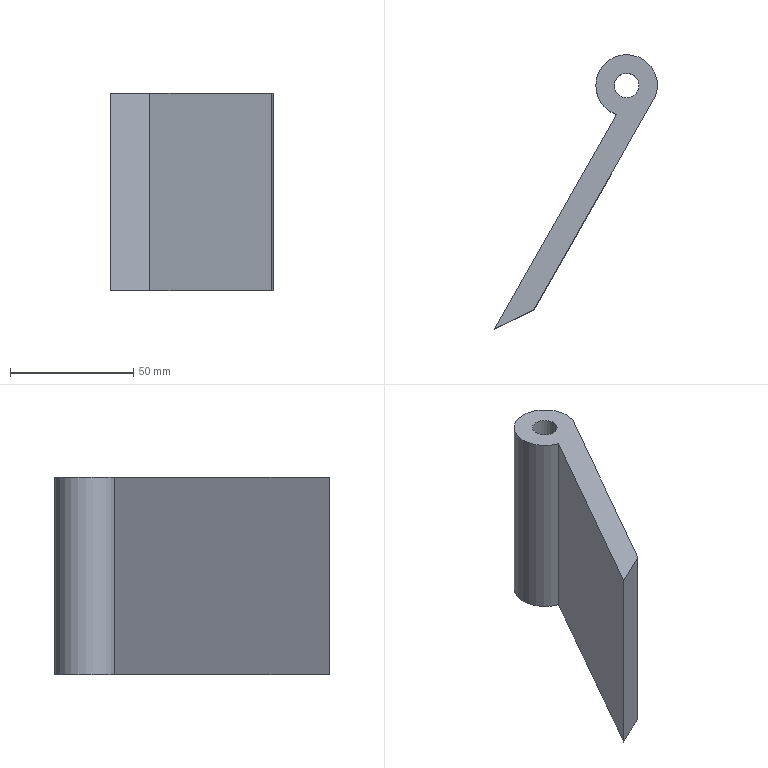Component | SolidWorks | Scraper-1 | 1 solid | 8 faces | box 66.03 x 111.24 x 80 mm | volume 109419 mm3 | plane 5 | cylinder 3 | commonest cylinder face diameters 10 x2 25 x1
build123d program:
from build123d import *

# Parameters (mm, degrees)
SKETCH1_R           = 5
BOSS_EXTRUDE1_DEPTH = 80


with BuildPart() as part:
    # Sketch1 → Boss-Extrude1 (new body)
    with BuildSketch(Plane(origin=(0, 0, 0), x_dir=(0, 0, -1), z_dir=(1, 0, 0))):
        with BuildLine():
            Line((-12.5, 0), (5.81, -98.31))
            Line((5.81, -98.31), (18.31, -110.81))
            Line((18.31, -110.81), (0, -12.5))
            ThreePointArc((0, -12.5), (8.839, 8.839), (-12.5, 0))
        make_face()
        Circle(SKETCH1_R, mode=Mode.SUBTRACT)
    extrude(amount=BOSS_EXTRUDE1_DEPTH)


solid = part.part

# Placed as in the assembly
solid = solid.moved(Location((504.241, -232.715, 1598.724), (90, 70.919, -90)))
STEP:
#1=COLOUR_RGB('',0.7922,0.8196,0.9333);
#2=FILL_AREA_STYLE_COLOUR('',#1);
#3=FILL_AREA_STYLE('',(#2));
#4=SURFACE_STYLE_FILL_AREA(#3);
#5=SURFACE_SIDE_STYLE('',(#4));
#6=SURFACE_STYLE_USAGE(.BOTH.,#5);
#7=PRESENTATION_STYLE_ASSIGNMENT((#6));
#8=CARTESIAN_POINT('',(20.038,-9.226,59.792));
#9=VERTEX_POINT('',#8);
#10=CARTESIAN_POINT('',(19.666,-9.098,59.792));
#11=VERTEX_POINT('',#10);
#12=CARTESIAN_POINT('',(19.852,-9.162,59.792));
#13=DIRECTION('',(-0.,-0.,-1.));
#14=DIRECTION('',(-0.9451,0.3269,0.));
#15=AXIS2_PLACEMENT_3D('',#12,#13,#14);
#16=CIRCLE('',#15,0.1969);
#17=EDGE_CURVE('',#9,#11,#16,.T.);
#18=ORIENTED_EDGE('',*,*,#17,.T.);
#19=CARTESIAN_POINT('',(19.666,-9.098,62.942));
#20=VERTEX_POINT('',#19);
#21=CARTESIAN_POINT('',(19.666,-9.098,59.792));
#22=DIRECTION('',(0.,0.,1.));
#23=VECTOR('',#22,39.37);
#24=LINE('',#21,#23);
#25=EDGE_CURVE('',#11,#20,#24,.T.);
#26=ORIENTED_EDGE('',*,*,#25,.T.);
#27=CARTESIAN_POINT('',(20.038,-9.226,62.942));
#28=VERTEX_POINT('',#27);
#29=CARTESIAN_POINT('',(19.852,-9.162,62.942));
#30=DIRECTION('',(-0.,-0.,-1.));
#31=DIRECTION('',(-0.9451,0.3269,0.));
#32=AXIS2_PLACEMENT_3D('',#29,#30,#31);
#33=CIRCLE('',#32,0.1969);
#34=EDGE_CURVE('',#28,#20,#33,.T.);
#35=ORIENTED_EDGE('',*,*,#34,.F.);
#36=CARTESIAN_POINT('',(20.038,-9.226,59.792));
#37=DIRECTION('',(0.,0.,1.));
#38=VECTOR('',#37,39.37);
#39=LINE('',#36,#38);
#40=EDGE_CURVE('',#9,#28,#39,.T.);
#41=ORIENTED_EDGE('',*,*,#40,.F.);
#42=EDGE_LOOP('',(#18,#26,#35,#41));
#43=FACE_OUTER_BOUND('',#42,.T.);
#44=CARTESIAN_POINT('',(19.852,-9.162,59.792));
#45=DIRECTION('',(0.,0.,1.));
#46=DIRECTION('',(0.9451,-0.3269,0.));
#47=AXIS2_PLACEMENT_3D('',#44,#45,#46);
#48=CYLINDRICAL_SURFACE('',#47,0.1969);
#49=ADVANCED_FACE('',(#43),#48,.F.);
#50=CARTESIAN_POINT('',(19.691,-9.627,59.792));
#51=VERTEX_POINT('',#50);
#52=CARTESIAN_POINT('',(20.317,-9.323,59.792));
#53=VERTEX_POINT('',#52);
#54=CARTESIAN_POINT('',(19.852,-9.162,59.792));
#55=DIRECTION('',(-0.,-0.,-1.));
#56=DIRECTION('',(-0.9451,0.3269,0.));
#57=AXIS2_PLACEMENT_3D('',#54,#55,#56);
#58=CIRCLE('',#57,0.4921);
#59=EDGE_CURVE('',#51,#53,#58,.T.);
#60=ORIENTED_EDGE('',*,*,#59,.T.);
#61=CARTESIAN_POINT('',(18.371,-12.745,59.792));
#62=VERTEX_POINT('',#61);
#63=CARTESIAN_POINT('',(20.317,-9.323,59.792));
#64=DIRECTION('',(-0.4944,-0.8692,0.));
#65=VECTOR('',#64,39.37);
#66=LINE('',#63,#65);
#67=EDGE_CURVE('',#53,#62,#66,.T.);
#68=ORIENTED_EDGE('',*,*,#67,.T.);
#69=CARTESIAN_POINT('',(17.745,-13.049,59.792));
#70=VERTEX_POINT('',#69);
#71=CARTESIAN_POINT('',(18.371,-12.745,59.792));
#72=DIRECTION('',(-0.8994,-0.4371,0.));
#73=VECTOR('',#72,39.37);
#74=LINE('',#71,#73);
#75=EDGE_CURVE('',#62,#70,#74,.T.);
#76=ORIENTED_EDGE('',*,*,#75,.T.);
#77=CARTESIAN_POINT('',(17.745,-13.049,59.792));
#78=DIRECTION('',(0.4944,0.8692,-0.));
#79=VECTOR('',#78,39.37);
#80=LINE('',#77,#79);
#81=EDGE_CURVE('',#70,#51,#80,.T.);
#82=ORIENTED_EDGE('',*,*,#81,.T.);
#83=EDGE_LOOP('',(#60,#68,#76,#82));
#84=FACE_OUTER_BOUND('',#83,.T.);
#85=ORIENTED_EDGE('',*,*,#17,.F.);
#86=CARTESIAN_POINT('',(19.852,-9.162,59.792));
#87=DIRECTION('',(-0.,-0.,-1.));
#88=DIRECTION('',(-0.9451,0.3269,0.));
#89=AXIS2_PLACEMENT_3D('',#86,#87,#88);
#90=CIRCLE('',#89,0.1969);
#91=EDGE_CURVE('',#11,#9,#90,.T.);
#92=ORIENTED_EDGE('',*,*,#91,.F.);
#93=EDGE_LOOP('',(#85,#92));
#94=FACE_BOUND('',#93,.T.);
#95=CARTESIAN_POINT('',(19.852,-9.162,59.792));
#96=DIRECTION('',(-0.,-0.,-1.));
#97=DIRECTION('',(-0.9451,0.3269,0.));
#98=AXIS2_PLACEMENT_3D('',#95,#96,#97);
#99=PLANE('',#98);
#100=ADVANCED_FACE('',(#84,#94),#99,.T.);
#101=CARTESIAN_POINT('',(19.691,-9.627,62.942));
#102=VERTEX_POINT('',#101);
#103=CARTESIAN_POINT('',(20.317,-9.323,62.942));
#104=VERTEX_POINT('',#103);
#105=CARTESIAN_POINT('',(19.852,-9.162,62.942));
#106=DIRECTION('',(-0.,-0.,-1.));
#107=DIRECTION('',(-0.9451,0.3269,0.));
#108=AXIS2_PLACEMENT_3D('',#105,#106,#107);
#109=CIRCLE('',#108,0.4921);
#110=EDGE_CURVE('',#102,#104,#109,.T.);
#111=ORIENTED_EDGE('',*,*,#110,.F.);
#112=CARTESIAN_POINT('',(17.745,-13.049,62.942));
#113=VERTEX_POINT('',#112);
#114=CARTESIAN_POINT('',(17.745,-13.049,62.942));
#115=DIRECTION('',(0.4944,0.8692,-0.));
#116=VECTOR('',#115,39.37);
#117=LINE('',#114,#116);
#118=EDGE_CURVE('',#113,#102,#117,.T.);
#119=ORIENTED_EDGE('',*,*,#118,.F.);
#120=CARTESIAN_POINT('',(18.371,-12.745,62.942));
#121=VERTEX_POINT('',#120);
#122=CARTESIAN_POINT('',(18.371,-12.745,62.942));
#123=DIRECTION('',(-0.8994,-0.4371,0.));
#124=VECTOR('',#123,39.37);
#125=LINE('',#122,#124);
#126=EDGE_CURVE('',#121,#113,#125,.T.);
#127=ORIENTED_EDGE('',*,*,#126,.F.);
#128=CARTESIAN_POINT('',(20.317,-9.323,62.942));
#129=DIRECTION('',(-0.4944,-0.8692,0.));
#130=VECTOR('',#129,39.37);
#131=LINE('',#128,#130);
#132=EDGE_CURVE('',#104,#121,#131,.T.);
#133=ORIENTED_EDGE('',*,*,#132,.F.);
#134=EDGE_LOOP('',(#111,#119,#127,#133));
#135=FACE_OUTER_BOUND('',#134,.T.);
#136=ORIENTED_EDGE('',*,*,#34,.T.);
#137=CARTESIAN_POINT('',(19.852,-9.162,62.942));
#138=DIRECTION('',(-0.,-0.,-1.));
#139=DIRECTION('',(-0.9451,0.3269,0.));
#140=AXIS2_PLACEMENT_3D('',#137,#138,#139);
#141=CIRCLE('',#140,0.1969);
#142=EDGE_CURVE('',#20,#28,#141,.T.);
#143=ORIENTED_EDGE('',*,*,#142,.T.);
#144=EDGE_LOOP('',(#136,#143));
#145=FACE_BOUND('',#144,.T.);
#146=CARTESIAN_POINT('',(19.852,-9.162,62.942));
#147=DIRECTION('',(-0.,-0.,-1.));
#148=DIRECTION('',(-0.9451,0.3269,0.));
#149=AXIS2_PLACEMENT_3D('',#146,#147,#148);
#150=PLANE('',#149);
#151=ADVANCED_FACE('',(#135,#145),#150,.F.);
#152=ORIENTED_EDGE('',*,*,#110,.T.);
#153=CARTESIAN_POINT('',(20.317,-9.323,59.792));
#154=DIRECTION('',(0.,0.,1.));
#155=VECTOR('',#154,39.37);
#156=LINE('',#153,#155);
#157=EDGE_CURVE('',#53,#104,#156,.T.);
#158=ORIENTED_EDGE('',*,*,#157,.F.);
#159=ORIENTED_EDGE('',*,*,#59,.F.);
#160=CARTESIAN_POINT('',(19.691,-9.627,59.792));
#161=DIRECTION('',(0.,0.,1.));
#162=VECTOR('',#161,39.37);
#163=LINE('',#160,#162);
#164=EDGE_CURVE('',#51,#102,#163,.T.);
#165=ORIENTED_EDGE('',*,*,#164,.T.);
#166=EDGE_LOOP('',(#152,#158,#159,#165));
#167=FACE_OUTER_BOUND('',#166,.T.);
#168=CARTESIAN_POINT('',(19.852,-9.162,59.792));
#169=DIRECTION('',(0.,0.,1.));
#170=DIRECTION('',(0.9451,-0.3269,0.));
#171=AXIS2_PLACEMENT_3D('',#168,#169,#170);
#172=CYLINDRICAL_SURFACE('',#171,0.4921);
#173=ADVANCED_FACE('',(#167),#172,.T.);
#174=ORIENTED_EDGE('',*,*,#132,.T.);
#175=CARTESIAN_POINT('',(18.371,-12.745,59.792));
#176=DIRECTION('',(0.,0.,1.));
#177=VECTOR('',#176,39.37);
#178=LINE('',#175,#177);
#179=EDGE_CURVE('',#62,#121,#178,.T.);
#180=ORIENTED_EDGE('',*,*,#179,.F.);
#181=ORIENTED_EDGE('',*,*,#67,.F.);
#182=ORIENTED_EDGE('',*,*,#157,.T.);
#183=EDGE_LOOP('',(#174,#180,#181,#182));
#184=FACE_OUTER_BOUND('',#183,.T.);
#185=CARTESIAN_POINT('',(20.317,-9.323,59.792));
#186=DIRECTION('',(-0.8692,0.4944,0.));
#187=DIRECTION('',(0.4944,0.8692,-0.));
#188=AXIS2_PLACEMENT_3D('',#185,#186,#187);
#189=PLANE('',#188);
#190=ADVANCED_FACE('',(#184),#189,.F.);
#191=ORIENTED_EDGE('',*,*,#126,.T.);
#192=CARTESIAN_POINT('',(17.745,-13.049,59.792));
#193=DIRECTION('',(0.,0.,1.));
#194=VECTOR('',#193,39.37);
#195=LINE('',#192,#194);
#196=EDGE_CURVE('',#70,#113,#195,.T.);
#197=ORIENTED_EDGE('',*,*,#196,.F.);
#198=ORIENTED_EDGE('',*,*,#75,.F.);
#199=ORIENTED_EDGE('',*,*,#179,.T.);
#200=EDGE_LOOP('',(#191,#197,#198,#199));
#201=FACE_OUTER_BOUND('',#200,.T.);
#202=CARTESIAN_POINT('',(18.371,-12.745,59.792));
#203=DIRECTION('',(-0.4371,0.8994,-0.));
#204=DIRECTION('',(0.8994,0.4371,-0.));
#205=AXIS2_PLACEMENT_3D('',#202,#203,#204);
#206=PLANE('',#205);
#207=ADVANCED_FACE('',(#201),#206,.F.);
#208=ORIENTED_EDGE('',*,*,#118,.T.);
#209=ORIENTED_EDGE('',*,*,#164,.F.);
#210=ORIENTED_EDGE('',*,*,#81,.F.);
#211=ORIENTED_EDGE('',*,*,#196,.T.);
#212=EDGE_LOOP('',(#208,#209,#210,#211));
#213=FACE_OUTER_BOUND('',#212,.T.);
#214=CARTESIAN_POINT('',(17.745,-13.049,59.792));
#215=DIRECTION('',(0.8692,-0.4944,-0.));
#216=DIRECTION('',(-0.4944,-0.8692,0.));
#217=AXIS2_PLACEMENT_3D('',#214,#215,#216);
#218=PLANE('',#217);
#219=ADVANCED_FACE('',(#213),#218,.F.);
#220=ORIENTED_EDGE('',*,*,#25,.F.);
#221=ORIENTED_EDGE('',*,*,#91,.T.);
#222=ORIENTED_EDGE('',*,*,#40,.T.);
#223=ORIENTED_EDGE('',*,*,#142,.F.);
#224=EDGE_LOOP('',(#220,#221,#222,#223));
#225=FACE_OUTER_BOUND('',#224,.T.);
#226=CARTESIAN_POINT('',(19.852,-9.162,59.792));
#227=DIRECTION('',(0.,0.,1.));
#228=DIRECTION('',(0.9451,-0.3269,0.));
#229=AXIS2_PLACEMENT_3D('',#226,#227,#228);
#230=CYLINDRICAL_SURFACE('',#229,0.1969);
#231=ADVANCED_FACE('',(#225),#230,.F.);
#232=CLOSED_SHELL('',(#49,#100,#151,#173,#190,#207,#219,#231));
#233=MANIFOLD_SOLID_BREP('',#232);
#234=STYLED_ITEM('',(#7),#233);
#235=PRESENTATION_LAYER_ASSIGNMENT('','',(#234));
#236=(LENGTH_UNIT()NAMED_UNIT(*)SI_UNIT($,.METRE.));
#237=LENGTH_MEASURE_WITH_UNIT(LENGTH_MEASURE(0.0254),#236);
#238=DIMENSIONAL_EXPONENTS(1.,0.,0.,0.,0.,0.,0.);
#239=(CONVERSION_BASED_UNIT('',#237)LENGTH_UNIT()NAMED_UNIT(#238));
#240=UNCERTAINTY_MEASURE_WITH_UNIT(LENGTH_MEASURE(0.00001),#239,'','');
#241=(NAMED_UNIT(*)PLANE_ANGLE_UNIT()SI_UNIT($,.RADIAN.));
#242=(NAMED_UNIT(*)SI_UNIT($,.STERADIAN.)SOLID_ANGLE_UNIT());
#243=(GEOMETRIC_REPRESENTATION_CONTEXT(3)GLOBAL_UNCERTAINTY_ASSIGNED_CONTEXT((#240))GLOBAL_UNIT_ASSIGNED_CONTEXT((#239,#241,#242))REPRESENTATION_CONTEXT('',''));
#244=MECHANICAL_DESIGN_GEOMETRIC_PRESENTATION_REPRESENTATION('',(#234),#243);
#245=CARTESIAN_POINT('',(0.,0.,0.));
#246=DIRECTION('',(0.,0.,1.));
#247=DIRECTION('',(1.,0.,0.));
#248=AXIS2_PLACEMENT_3D('',#245,#246,#247);
#249=(LENGTH_UNIT()NAMED_UNIT(*)SI_UNIT($,.METRE.));
#250=LENGTH_MEASURE_WITH_UNIT(LENGTH_MEASURE(0.0254),#249);
#251=DIMENSIONAL_EXPONENTS(1.,0.,0.,0.,0.,0.,0.);
#252=(CONVERSION_BASED_UNIT('',#250)LENGTH_UNIT()NAMED_UNIT(#251));
#253=UNCERTAINTY_MEASURE_WITH_UNIT(LENGTH_MEASURE(0.00001),#252,'','');
#254=(NAMED_UNIT(*)PLANE_ANGLE_UNIT()SI_UNIT($,.RADIAN.));
#255=(NAMED_UNIT(*)SI_UNIT($,.STERADIAN.)SOLID_ANGLE_UNIT());
#256=(GEOMETRIC_REPRESENTATION_CONTEXT(3)GLOBAL_UNCERTAINTY_ASSIGNED_CONTEXT((#253))GLOBAL_UNIT_ASSIGNED_CONTEXT((#252,#254,#255))REPRESENTATION_CONTEXT('',''));
#257=ADVANCED_BREP_SHAPE_REPRESENTATION('',(#233,#248),#256);